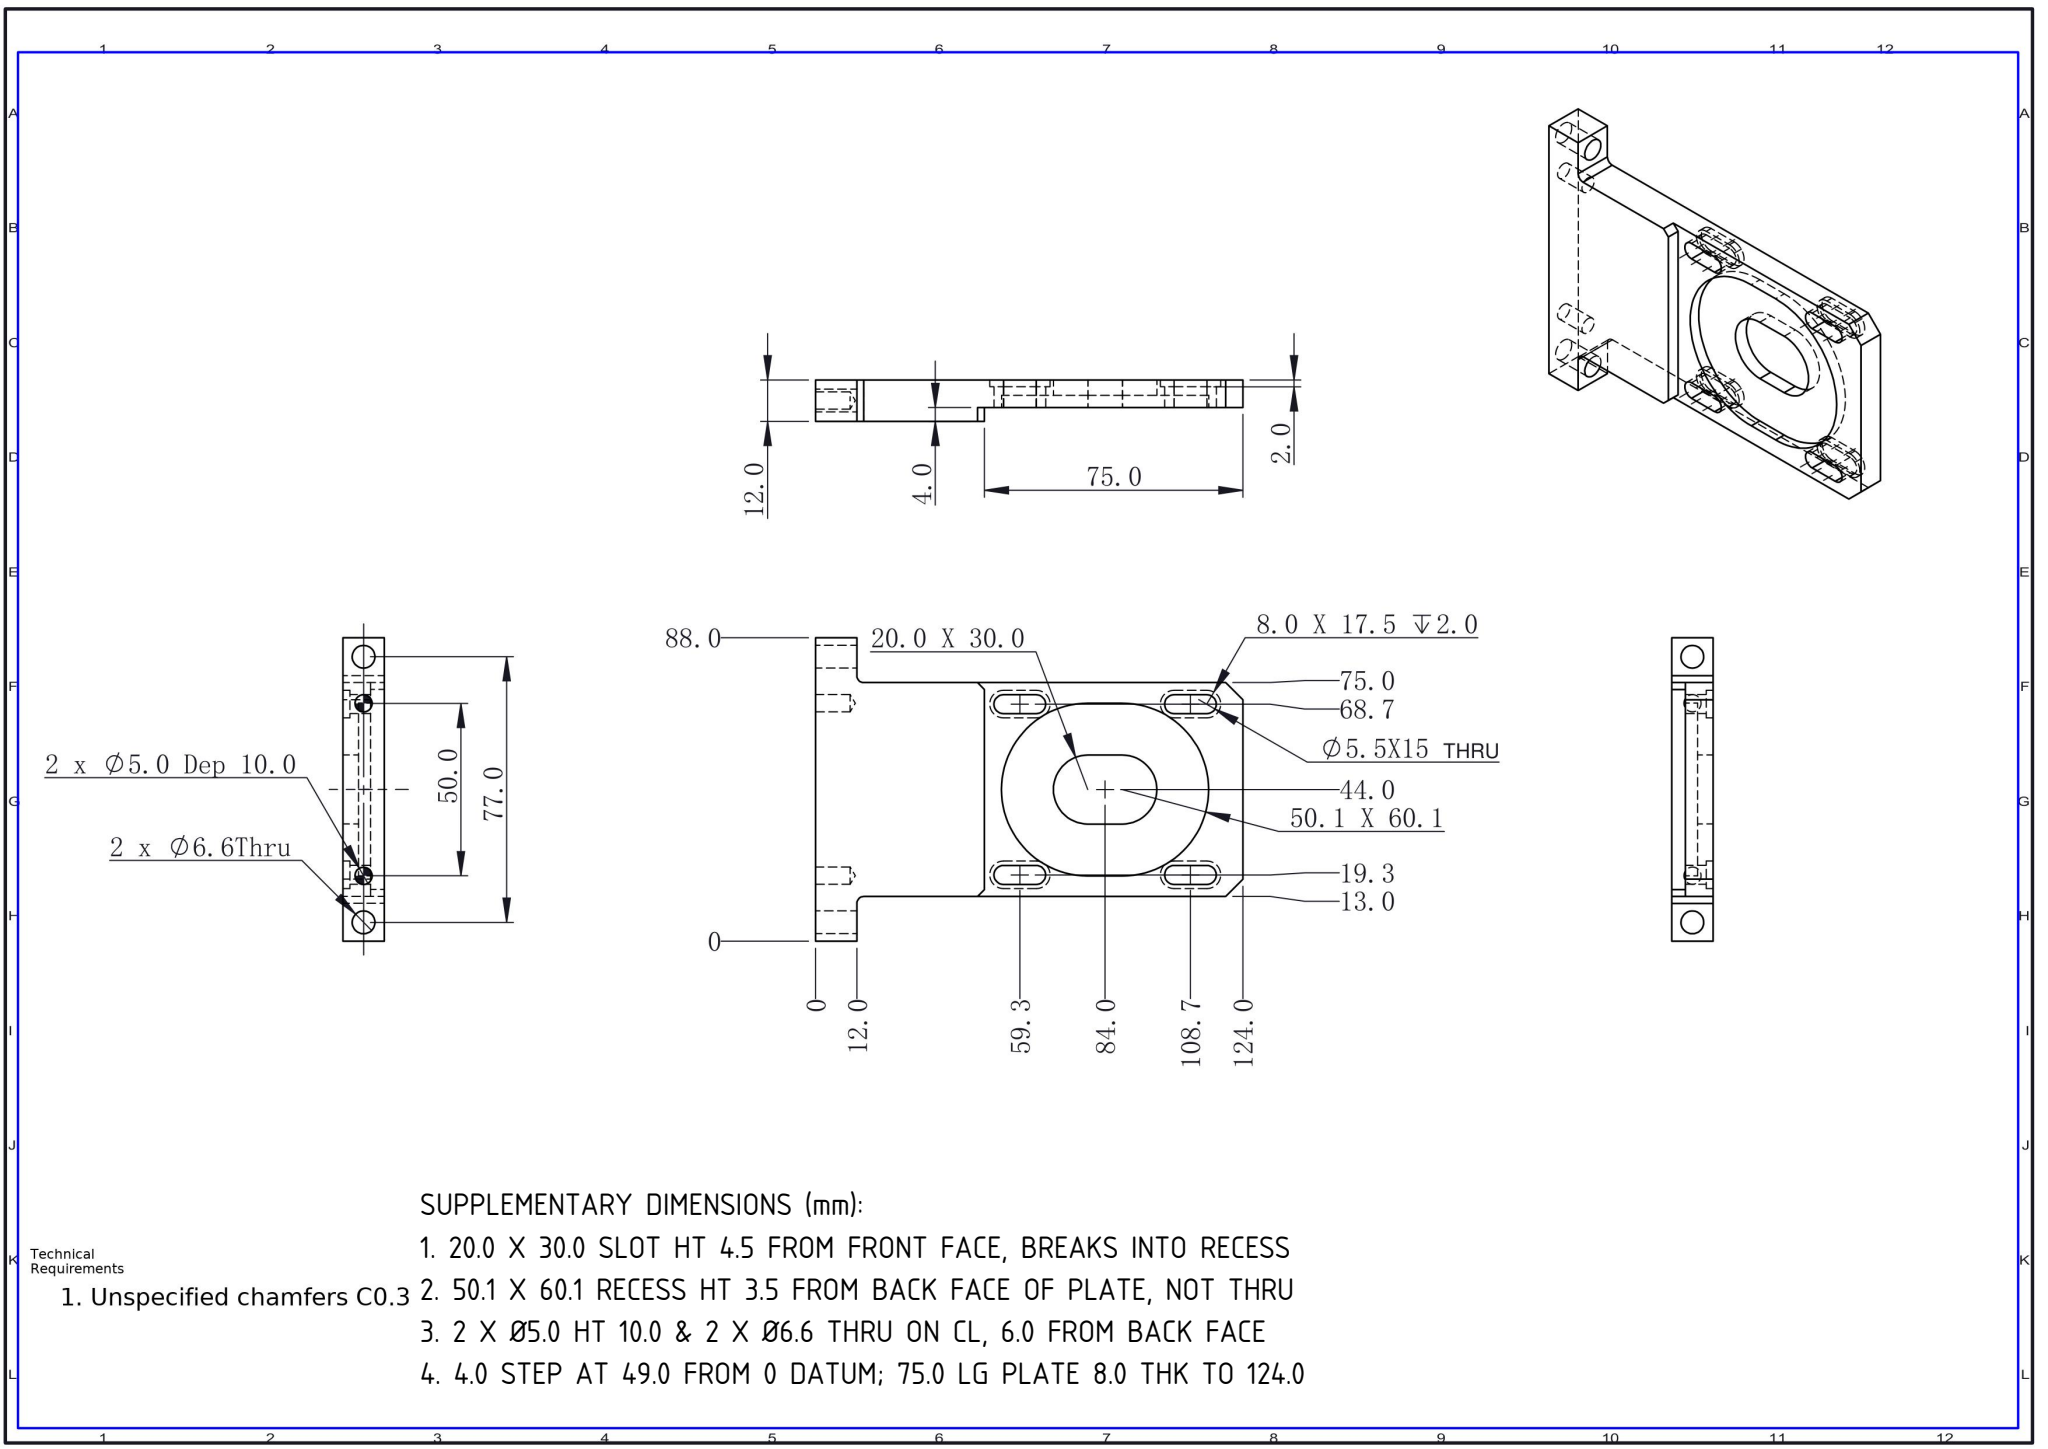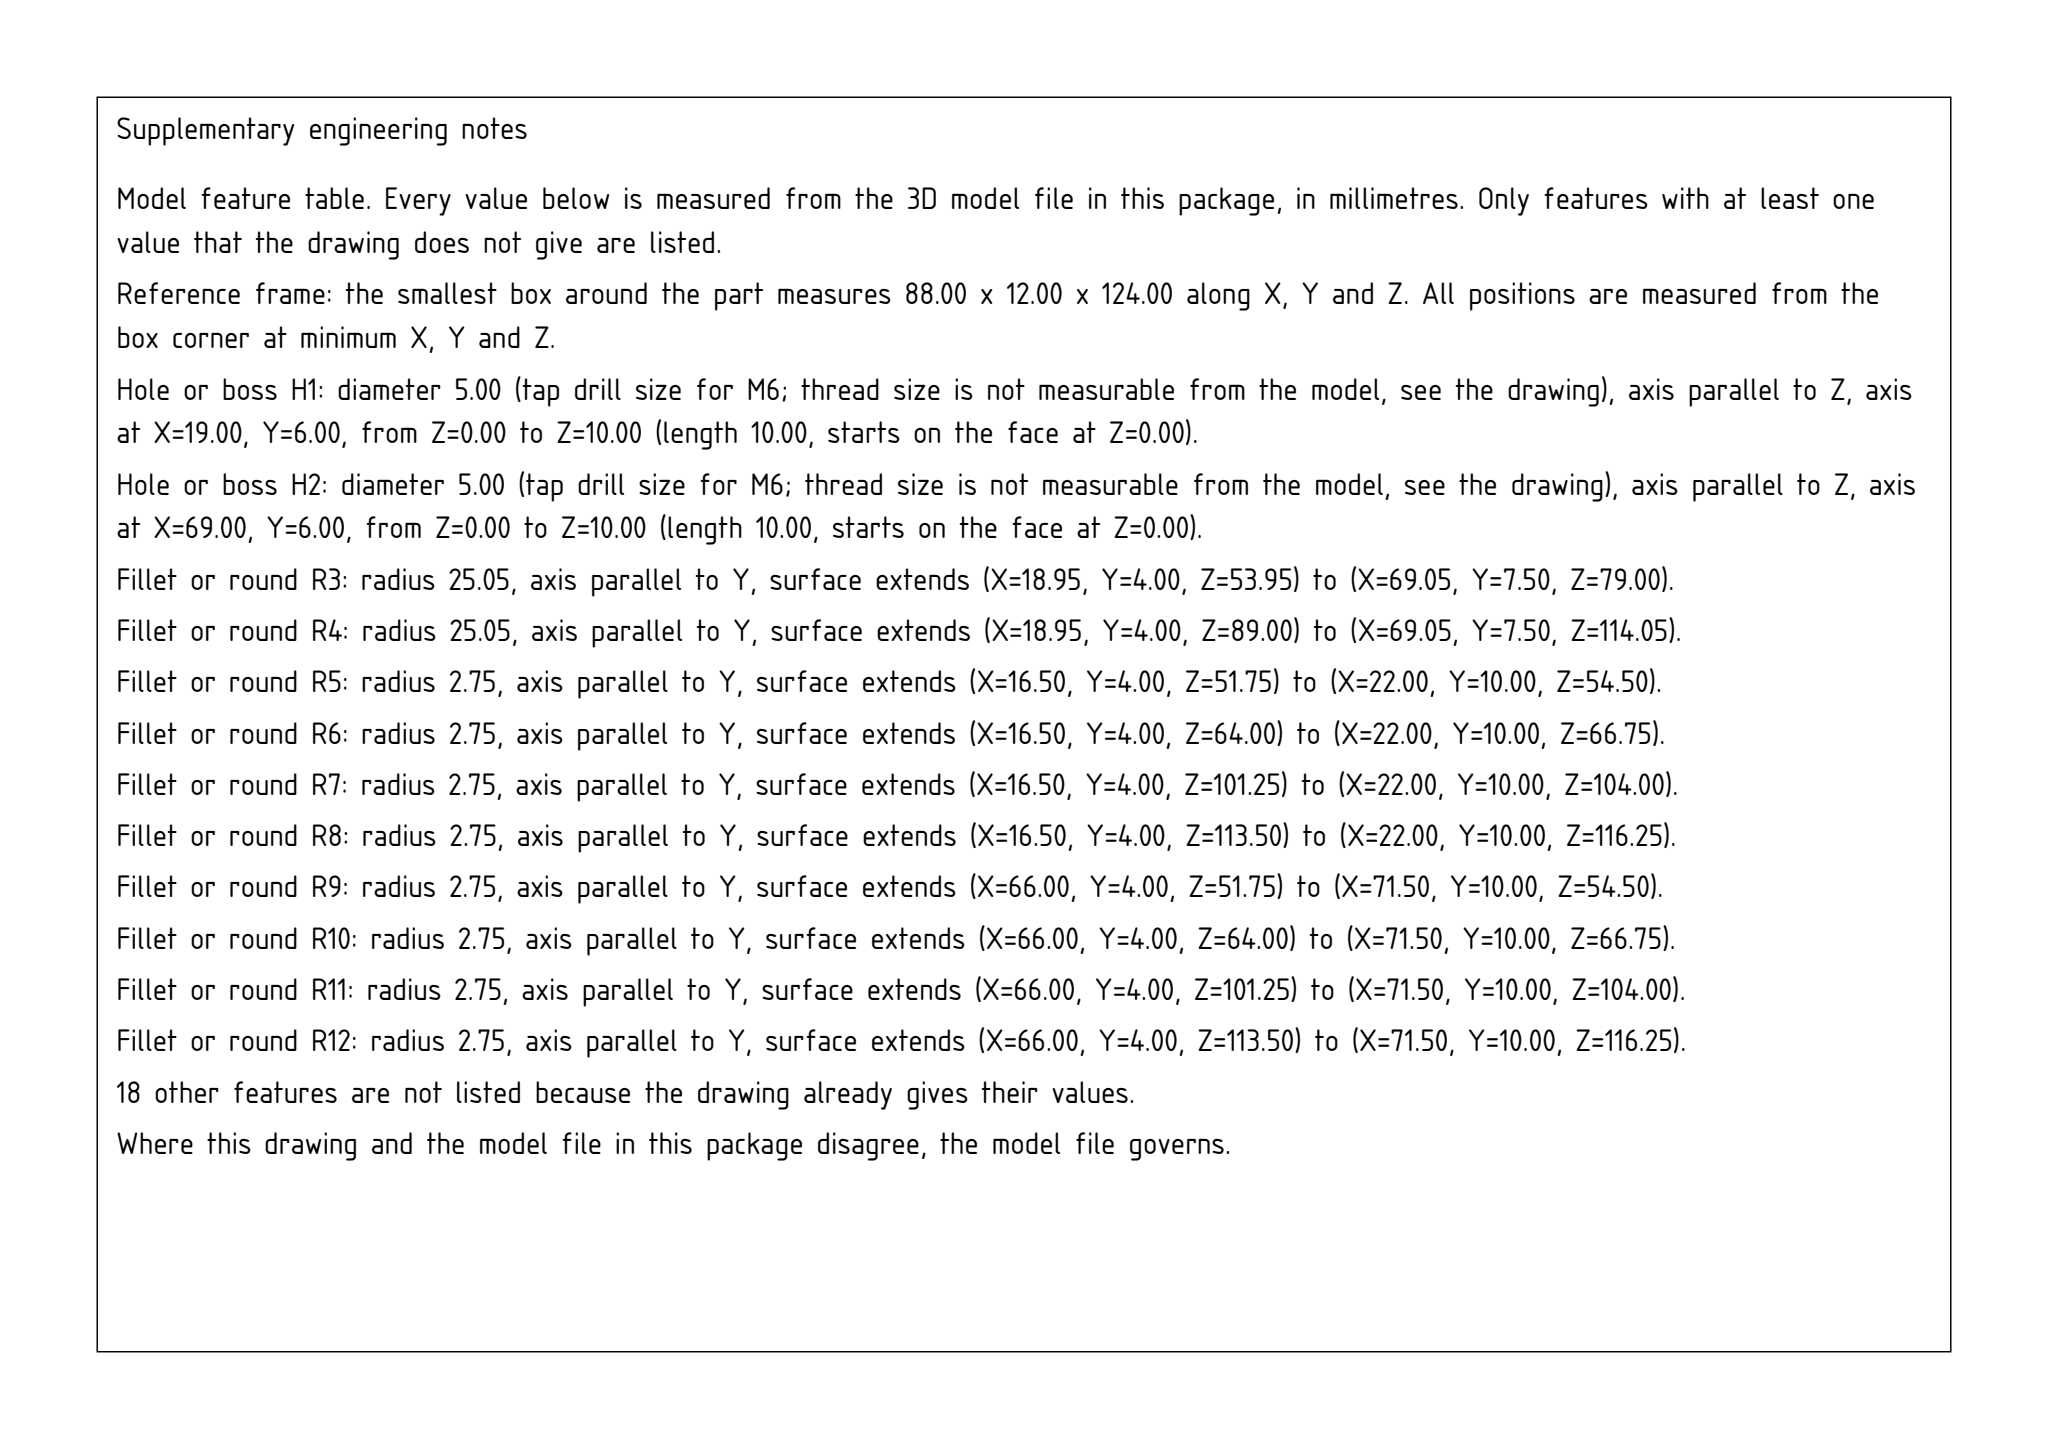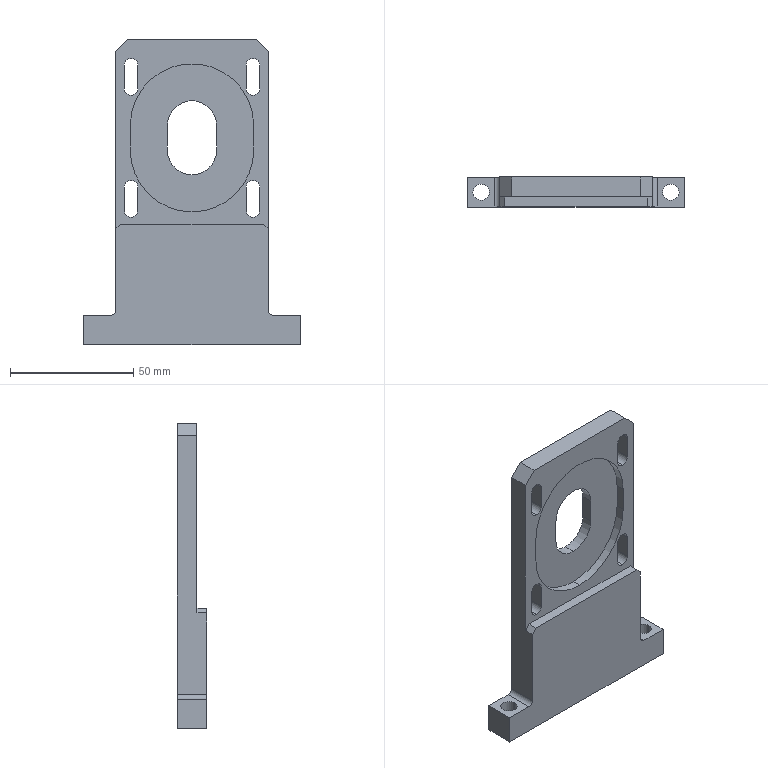Part | SolidWorks | mm | 1 solid | 85 faces | box 88 x 12 x 124 mm | volume 62170 mm3 | plane 41 | cylinder 40 | cone 4 | commonest cylinder face diameters 8 x12 5.5 x12 5 x4 6.6 x4 20 x3 50.1 x3 4 x2